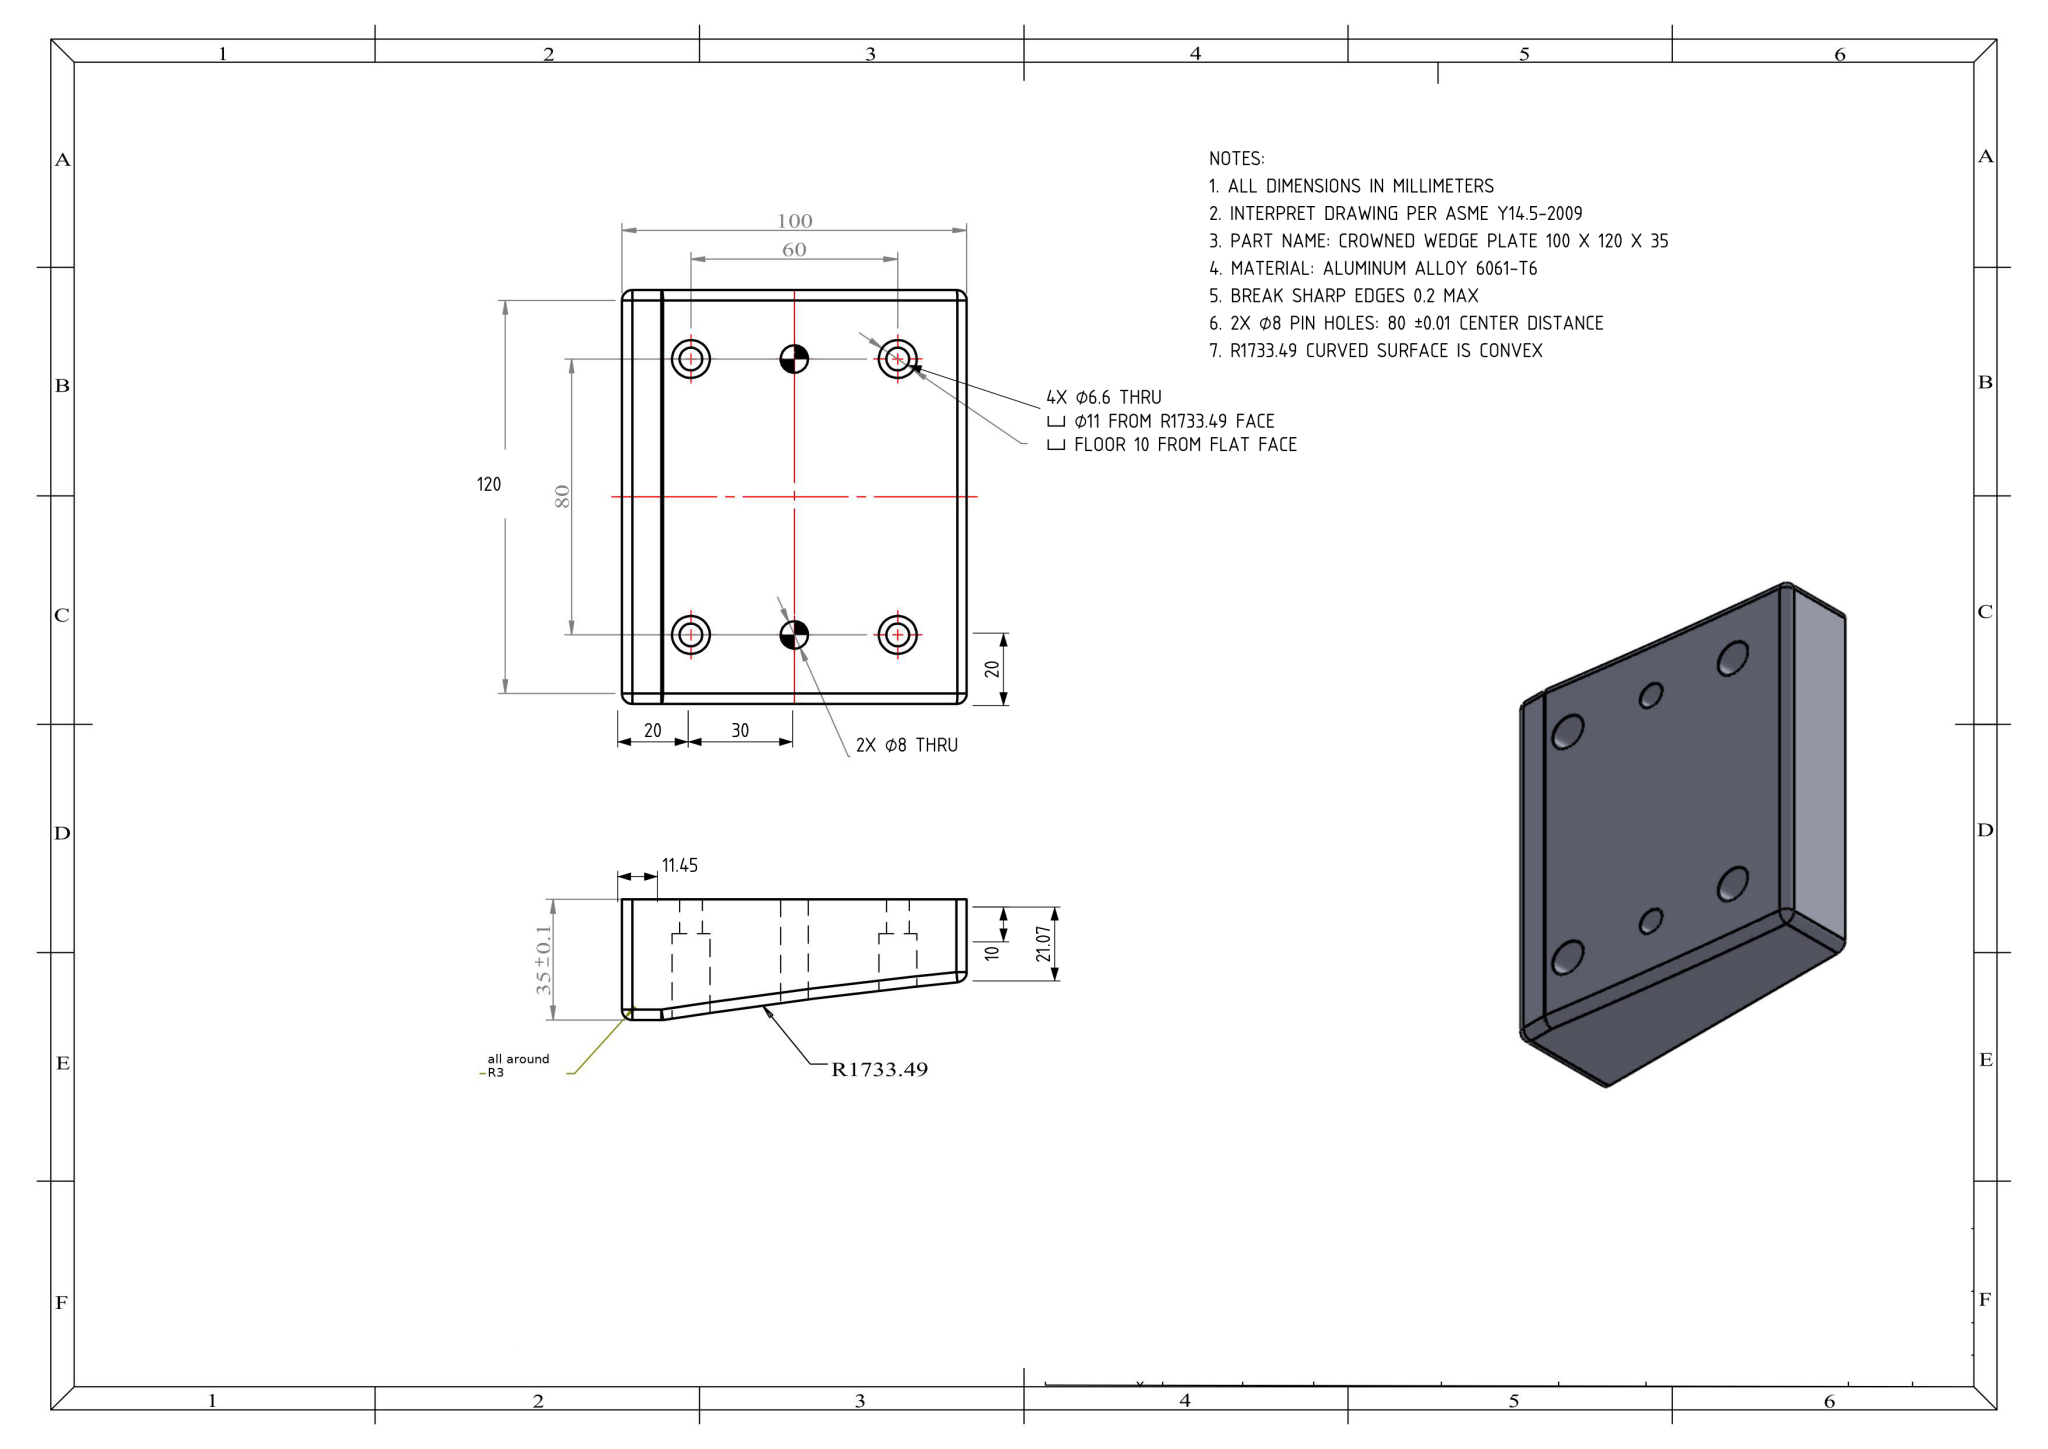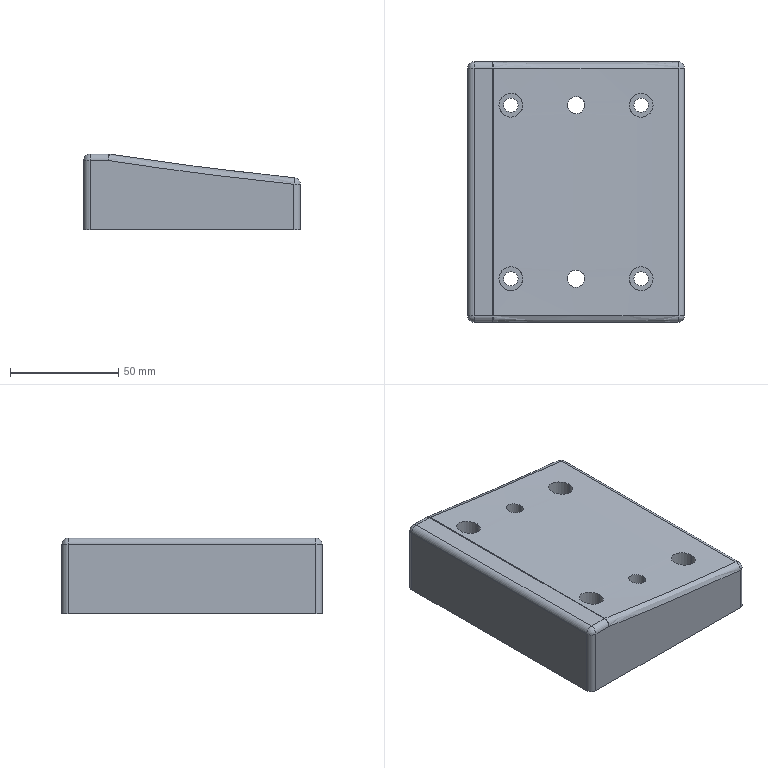Part | NX | mm | 1 solid | 48 faces | box 100 x 120 x 35 mm | volume 343569 mm3 | cylinder 29 | plane 10 | sphere 6 | spline 3 | commonest cylinder face diameters 6 x9 6.6 x8 11 x8 8 x4